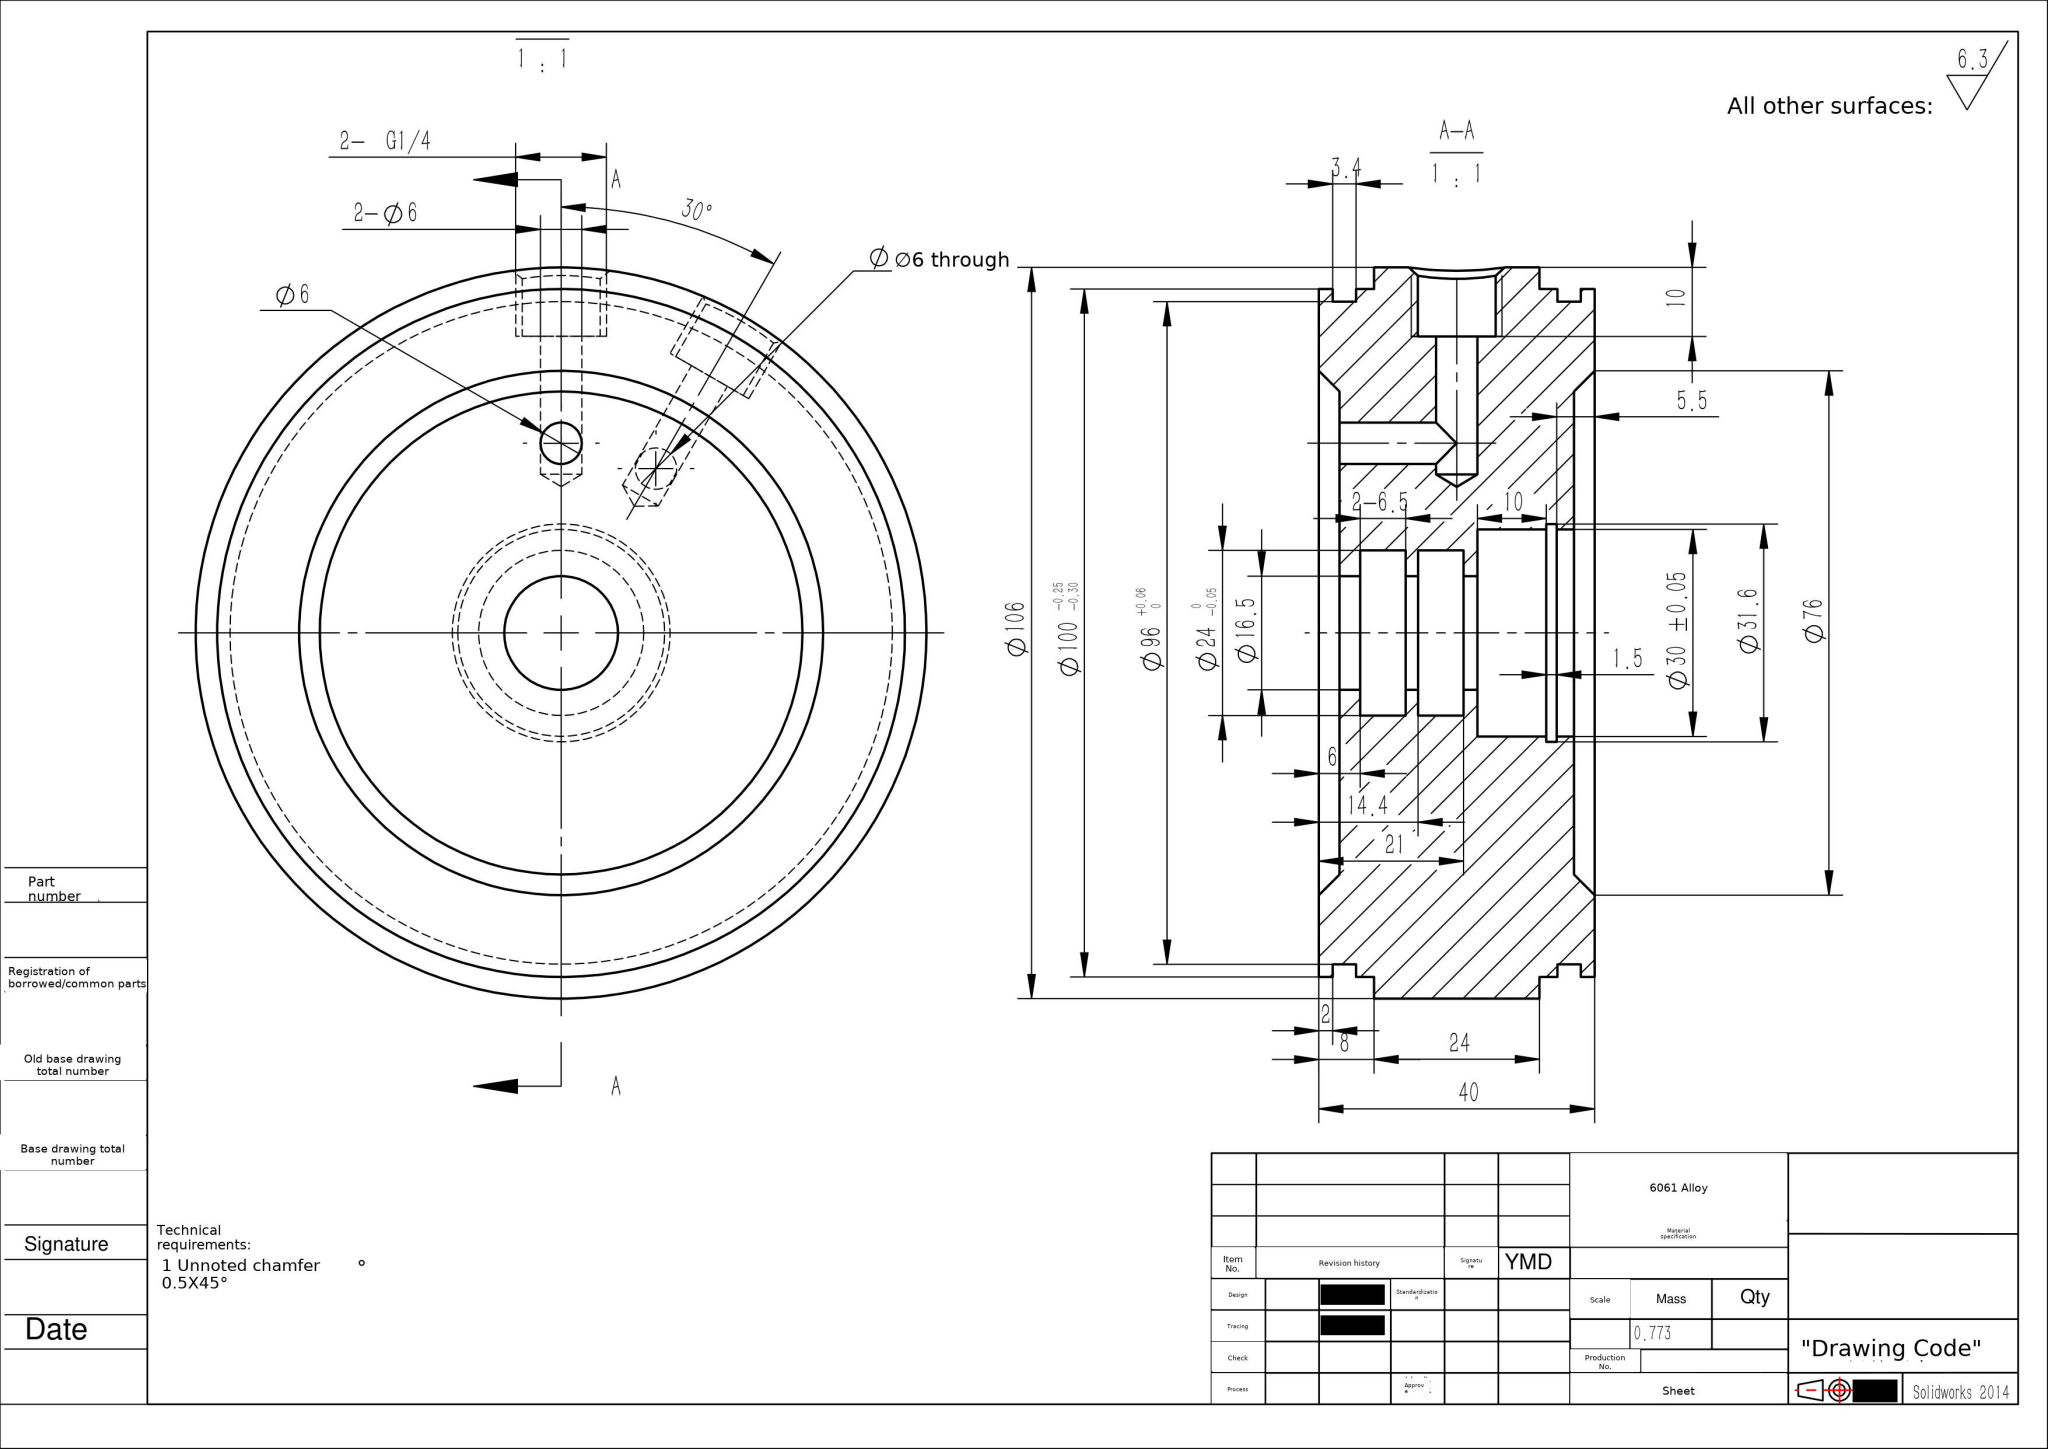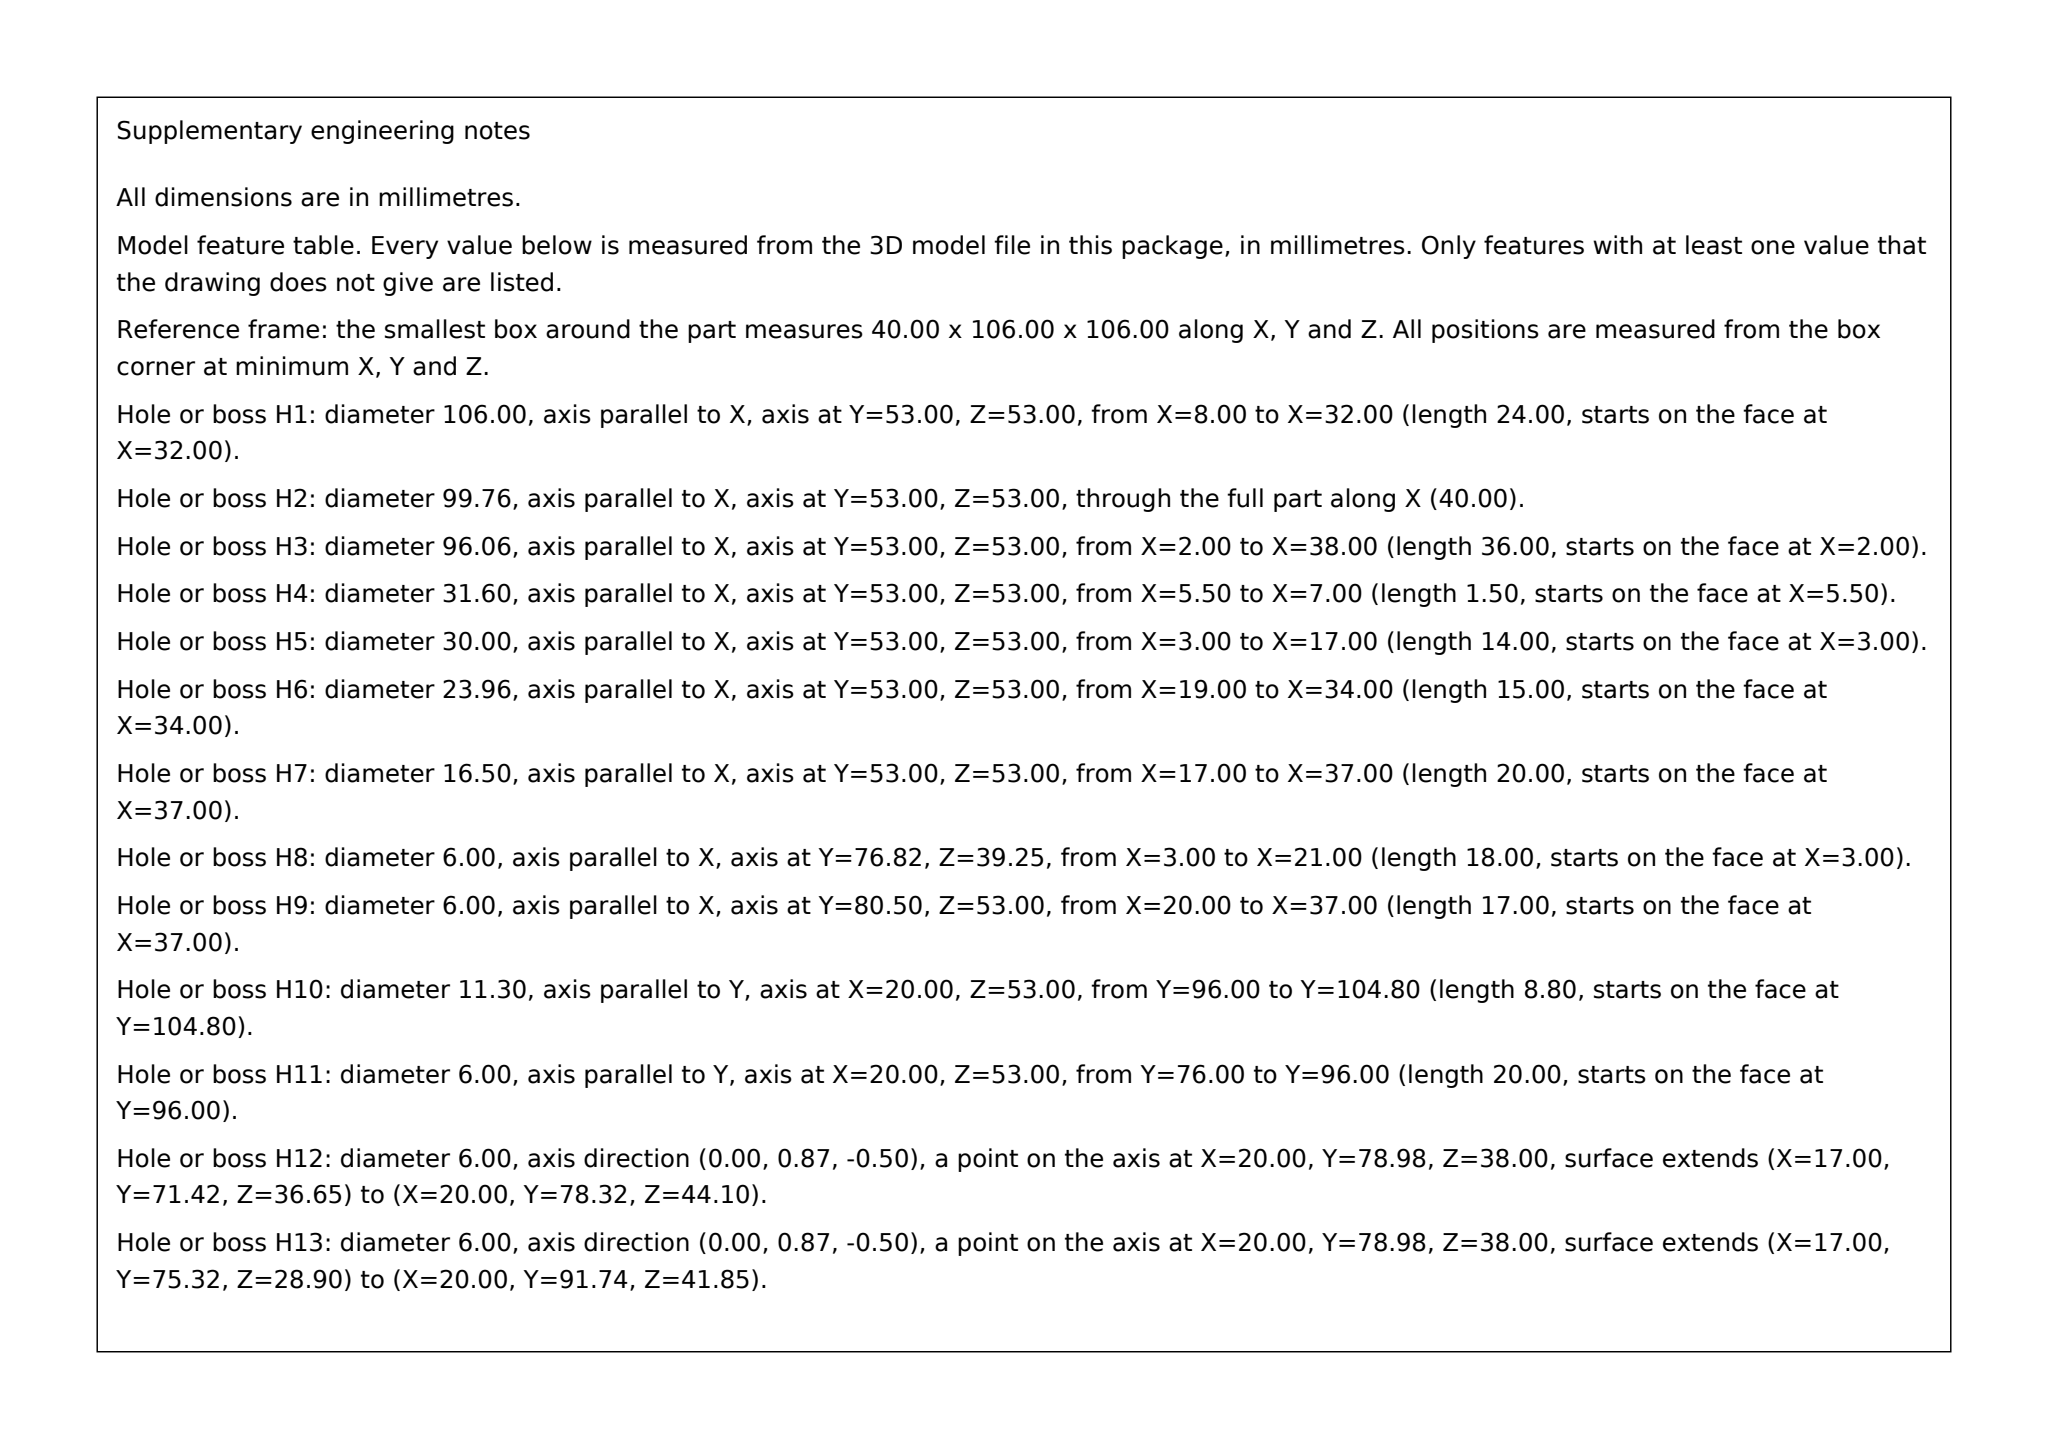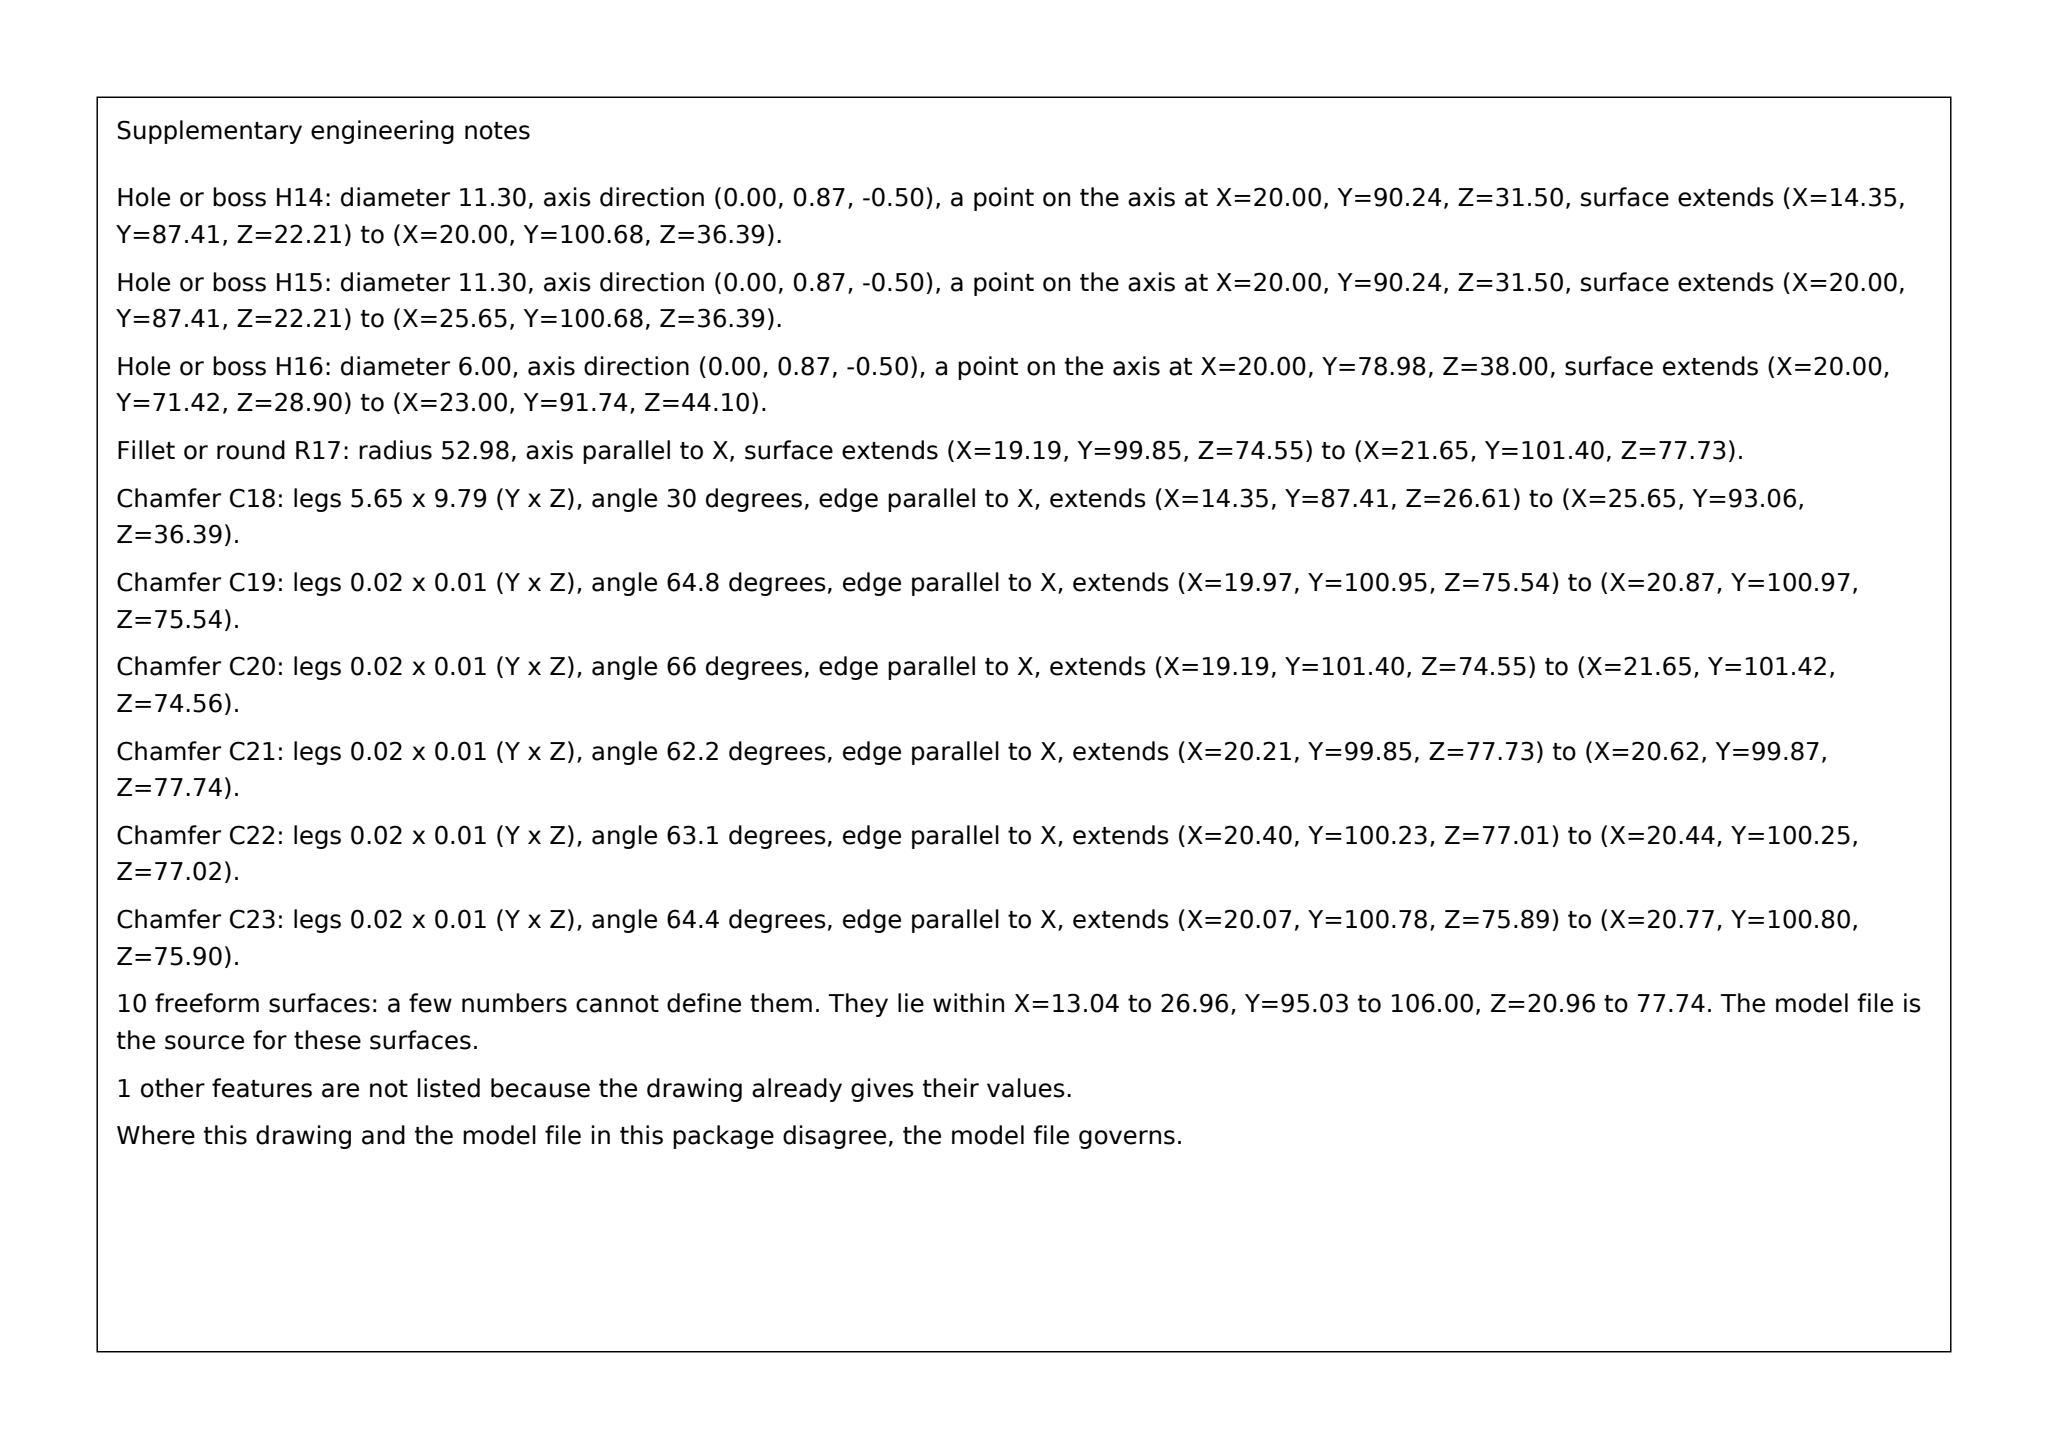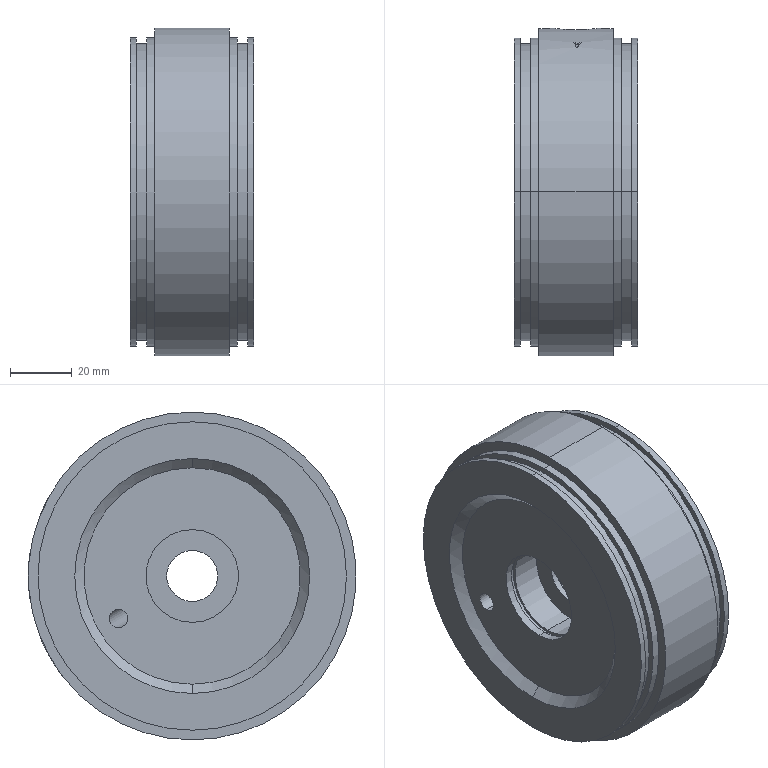Part | SolidWorks | mm | material 6061 Alloy | 1 solid | 93 faces | box 40 x 106 x 106 mm | volume 286407 mm3 | cylinder 48 | plane 27 | spline 10 | cone 8 | commonest cylinder face diameters 6 x12 99.75 x8 16.5 x6 11.3 x4 23.95 x4 96.06 x4 30 x4 106 x3